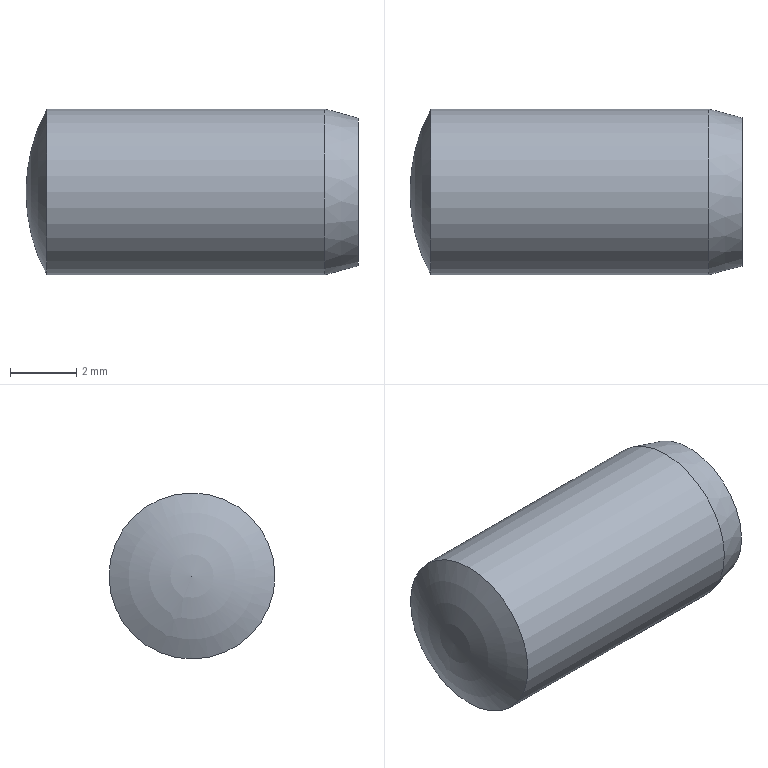Component | NX | CH3404_8-5_4 | 1 solid | 4 faces | box 10 x 5 x 5 mm | volume 188 mm3 | sphere 1 | plane 1 | cone 1 | cylinder 1 | commonest cylinder face diameters 5 x1
STEP:
#1=CARTESIAN_POINT('',(0.,0.,0.));
#2=DIRECTION('',(0.,0.,1.));
#3=DIRECTION('',(1.,0.,0.));
#4=AXIS2_PLACEMENT_3D('',#1,#2,#3);
#5=CARTESIAN_POINT('',(-39.37,0.9546,97.689));
#6=VERTEX_POINT('',#5);
#7=CARTESIAN_POINT('',(-39.37,-2.311,99.045));
#8=VERTEX_POINT('',#7);
#9=CARTESIAN_POINT('',(-39.37,0.,100.));
#10=DIRECTION('',(1.,0.,0.));
#11=DIRECTION('',(0.,-0.9242,-0.3818));
#12=AXIS2_PLACEMENT_3D('',#9,#10,#11);
#13=CIRCLE('',#12,2.5);
#14=CARTESIAN_POINT('',(-34.725,0.,100.));
#15=DIRECTION('',(1.,0.,0.));
#16=DIRECTION('',(-0.,0.3818,-0.9242));
#17=AXIS2_PLACEMENT_3D('',#14,#15,#16);
#18=SPHERICAL_SURFACE('',#17,5.275);
#19=CARTESIAN_POINT('',(-1.571,-1.077));
#20=CARTESIAN_POINT('',(-1.476,-1.077));
#21=CARTESIAN_POINT('',(-1.285,-1.077));
#22=CARTESIAN_POINT('',(-0.9996,-1.077));
#23=CARTESIAN_POINT('',(-0.714,-1.077));
#24=CARTESIAN_POINT('',(-0.4284,-1.077));
#25=CARTESIAN_POINT('',(-0.1428,-1.077));
#26=CARTESIAN_POINT('',(0.1428,-1.077));
#27=CARTESIAN_POINT('',(0.4284,-1.077));
#28=CARTESIAN_POINT('',(0.714,-1.077));
#29=CARTESIAN_POINT('',(0.9996,-1.077));
#30=CARTESIAN_POINT('',(1.285,-1.077));
#31=CARTESIAN_POINT('',(1.571,-1.077));
#32=CARTESIAN_POINT('',(1.856,-1.077));
#33=CARTESIAN_POINT('',(2.142,-1.077));
#34=CARTESIAN_POINT('',(2.428,-1.077));
#35=CARTESIAN_POINT('',(2.713,-1.077));
#36=CARTESIAN_POINT('',(2.999,-1.077));
#37=CARTESIAN_POINT('',(3.284,-1.077));
#38=CARTESIAN_POINT('',(3.57,-1.077));
#39=CARTESIAN_POINT('',(3.856,-1.077));
#40=CARTESIAN_POINT('',(4.141,-1.077));
#41=CARTESIAN_POINT('',(4.427,-1.077));
#42=CARTESIAN_POINT('',(4.617,-1.077));
#43=CARTESIAN_POINT('',(4.712,-1.077));
#44=B_SPLINE_CURVE_WITH_KNOTS('',3,(#19,#20,#21,#22,#23,#24,#25,#26,#27,#28,#29,#30,#31,#32,#33,#34,#35,#36,#37,#38,#39,#40,#41,#42,#43),.UNSPECIFIED.,.F.,.F.,(4,1,1,1,1,1,1,1,1,1,1,1,1,1,1,1,1,1,1,1,1,1,4),(0.,0.2856,0.5712,0.8568,1.142,1.428,1.714,1.999,2.285,2.57,2.856,3.142,3.427,3.713,3.998,4.284,4.57,4.855,5.141,5.426,5.712,5.998,6.283),.QUASI_UNIFORM_KNOTS.);
#45=(GEOMETRIC_REPRESENTATION_CONTEXT(2)PARAMETRIC_REPRESENTATION_CONTEXT()REPRESENTATION_CONTEXT('',''));
#46=DEFINITIONAL_REPRESENTATION('',(#44),#45);
#47=PCURVE('',#18,#46);
#48=CARTESIAN_POINT('',(-30.,0.,100.));
#49=DIRECTION('',(1.,0.,0.));
#50=DIRECTION('',(0.,-0.9242,-0.3818));
#51=AXIS2_PLACEMENT_3D('',#48,#49,#50);
#52=CYLINDRICAL_SURFACE('',#51,2.5);
#53=CARTESIAN_POINT('',(-0.,-9.37));
#54=DIRECTION('',(1.,0.));
#55=VECTOR('',#54,1.);
#56=LINE('',#53,#55);
#57=(GEOMETRIC_REPRESENTATION_CONTEXT(2)PARAMETRIC_REPRESENTATION_CONTEXT()REPRESENTATION_CONTEXT('',''));
#58=DEFINITIONAL_REPRESENTATION('',(#56),#57);
#59=PCURVE('',#52,#58);
#60=SURFACE_CURVE('',#13,(#47,#59),.PCURVE_S1.);
#61=EDGE_CURVE('',#6,#8,#60,.T.);
#62=ORIENTED_EDGE('',*,*,#61,.F.);
#63=CARTESIAN_POINT('',(-40.,-0.,100.));
#64=VERTEX_POINT('',#63);
#65=CARTESIAN_POINT('',(-40.,0.,100.));
#66=CARTESIAN_POINT('',(-40.,0.1989,99.519));
#67=CARTESIAN_POINT('',(-39.936,0.3978,99.037));
#68=CARTESIAN_POINT('',(-39.807,0.5927,98.565));
#69=CARTESIAN_POINT('',(-39.617,0.7795,98.113));
#70=CARTESIAN_POINT('',(-39.37,0.9546,97.689));
#71=B_SPLINE_CURVE_WITH_KNOTS('',5,(#65,#66,#67,#68,#69,#70),.UNSPECIFIED.,.F.,.F.,(6,6),(-1.571,-1.077),.PIECEWISE_BEZIER_KNOTS.);
#72=CARTESIAN_POINT('',(0.,0.));
#73=DIRECTION('',(0.,1.));
#74=VECTOR('',#73,1.);
#75=LINE('',#72,#74);
#76=(GEOMETRIC_REPRESENTATION_CONTEXT(2)PARAMETRIC_REPRESENTATION_CONTEXT()REPRESENTATION_CONTEXT('',''));
#77=DEFINITIONAL_REPRESENTATION('',(#75),#76);
#78=PCURVE('',#18,#77);
#79=CARTESIAN_POINT('',(6.283,0.));
#80=DIRECTION('',(0.,1.));
#81=VECTOR('',#80,1.);
#82=LINE('',#79,#81);
#83=(GEOMETRIC_REPRESENTATION_CONTEXT(2)PARAMETRIC_REPRESENTATION_CONTEXT()REPRESENTATION_CONTEXT('',''));
#84=DEFINITIONAL_REPRESENTATION('',(#82),#83);
#85=PCURVE('',#18,#84);
#86=SEAM_CURVE('',#71,(#78,#85),.PCURVE_S1.);
#87=EDGE_CURVE('',#64,#6,#86,.T.);
#88=ORIENTED_EDGE('',*,*,#87,.F.);
#89=ORIENTED_EDGE('',*,*,#87,.T.);
#90=CARTESIAN_POINT('',(-39.37,0.,100.));
#91=DIRECTION('',(1.,0.,0.));
#92=DIRECTION('',(0.,-0.9242,-0.3818));
#93=AXIS2_PLACEMENT_3D('',#90,#91,#92);
#94=CIRCLE('',#93,2.5);
#95=CARTESIAN_POINT('',(4.712,-1.077));
#96=CARTESIAN_POINT('',(4.808,-1.077));
#97=CARTESIAN_POINT('',(4.998,-1.077));
#98=CARTESIAN_POINT('',(5.284,-1.077));
#99=CARTESIAN_POINT('',(5.569,-1.077));
#100=CARTESIAN_POINT('',(5.855,-1.077));
#101=CARTESIAN_POINT('',(6.14,-1.077));
#102=CARTESIAN_POINT('',(6.426,-1.077));
#103=CARTESIAN_POINT('',(6.712,-1.077));
#104=CARTESIAN_POINT('',(6.997,-1.077));
#105=CARTESIAN_POINT('',(7.283,-1.077));
#106=CARTESIAN_POINT('',(7.568,-1.077));
#107=CARTESIAN_POINT('',(7.854,-1.077));
#108=CARTESIAN_POINT('',(8.14,-1.077));
#109=CARTESIAN_POINT('',(8.425,-1.077));
#110=CARTESIAN_POINT('',(8.711,-1.077));
#111=CARTESIAN_POINT('',(8.996,-1.077));
#112=CARTESIAN_POINT('',(9.282,-1.077));
#113=CARTESIAN_POINT('',(9.568,-1.077));
#114=CARTESIAN_POINT('',(9.853,-1.077));
#115=CARTESIAN_POINT('',(10.139,-1.077));
#116=CARTESIAN_POINT('',(10.424,-1.077));
#117=CARTESIAN_POINT('',(10.71,-1.077));
#118=CARTESIAN_POINT('',(10.9,-1.077));
#119=CARTESIAN_POINT('',(10.996,-1.077));
#120=B_SPLINE_CURVE_WITH_KNOTS('',3,(#95,#96,#97,#98,#99,#100,#101,#102,#103,#104,#105,#106,#107,#108,#109,#110,#111,#112,#113,#114,#115,#116,#117,#118,#119),.UNSPECIFIED.,.F.,.F.,(4,1,1,1,1,1,1,1,1,1,1,1,1,1,1,1,1,1,1,1,1,1,4),(0.,0.2856,0.5712,0.8568,1.142,1.428,1.714,1.999,2.285,2.57,2.856,3.142,3.427,3.713,3.998,4.284,4.57,4.855,5.141,5.426,5.712,5.998,6.283),.QUASI_UNIFORM_KNOTS.);
#121=(GEOMETRIC_REPRESENTATION_CONTEXT(2)PARAMETRIC_REPRESENTATION_CONTEXT()REPRESENTATION_CONTEXT('',''));
#122=DEFINITIONAL_REPRESENTATION('',(#120),#121);
#123=PCURVE('',#18,#122);
#124=CARTESIAN_POINT('',(0.,-9.37));
#125=DIRECTION('',(1.,0.));
#126=VECTOR('',#125,1.);
#127=LINE('',#124,#126);
#128=(GEOMETRIC_REPRESENTATION_CONTEXT(2)PARAMETRIC_REPRESENTATION_CONTEXT()REPRESENTATION_CONTEXT('',''));
#129=DEFINITIONAL_REPRESENTATION('',(#127),#128);
#130=PCURVE('',#52,#129);
#131=SURFACE_CURVE('',#94,(#123,#130),.PCURVE_S1.);
#132=EDGE_CURVE('',#8,#6,#131,.T.);
#133=ORIENTED_EDGE('',*,*,#132,.F.);
#134=EDGE_LOOP('',(#62,#88,#89,#133));
#135=FACE_BOUND('',#134,.T.);
#136=ADVANCED_FACE('',(#135),#18,.T.);
#137=CARTESIAN_POINT('',(-30.,-2.063,99.148));
#138=VERTEX_POINT('',#137);
#139=CARTESIAN_POINT('',(-30.,0.,100.));
#140=DIRECTION('',(1.,0.,0.));
#141=DIRECTION('',(0.,-0.9242,-0.3818));
#142=AXIS2_PLACEMENT_3D('',#139,#140,#141);
#143=CIRCLE('',#142,2.232);
#144=CARTESIAN_POINT('',(-30.,0.,100.));
#145=DIRECTION('',(1.,0.,0.));
#146=DIRECTION('',(0.,-0.9242,-0.3818));
#147=AXIS2_PLACEMENT_3D('',#144,#145,#146);
#148=PLANE('',#147);
#149=CARTESIAN_POINT('',(0.,-0.));
#150=DIRECTION('',(1.,0.));
#151=AXIS2_PLACEMENT_2D('',#149,#150);
#152=CIRCLE('',#151,2.232);
#153=(GEOMETRIC_REPRESENTATION_CONTEXT(2)PARAMETRIC_REPRESENTATION_CONTEXT()REPRESENTATION_CONTEXT('',''));
#154=DEFINITIONAL_REPRESENTATION('',(#152),#153);
#155=PCURVE('',#148,#154);
#156=CARTESIAN_POINT('',(-30.,0.,100.));
#157=DIRECTION('',(-1.,0.,0.));
#158=DIRECTION('',(0.,0.9242,0.3818));
#159=AXIS2_PLACEMENT_3D('',#156,#157,#158);
#160=CONICAL_SURFACE('',#159,2.232,0.2618);
#161=CARTESIAN_POINT('',(9.425,0.));
#162=DIRECTION('',(-1.,0.));
#163=VECTOR('',#162,1.);
#164=LINE('',#161,#163);
#165=(GEOMETRIC_REPRESENTATION_CONTEXT(2)PARAMETRIC_REPRESENTATION_CONTEXT()REPRESENTATION_CONTEXT('',''));
#166=DEFINITIONAL_REPRESENTATION('',(#164),#165);
#167=PCURVE('',#160,#166);
#168=SURFACE_CURVE('',#143,(#155,#167),.PCURVE_S1.);
#169=EDGE_CURVE('',#138,#138,#168,.T.);
#170=ORIENTED_EDGE('',*,*,#169,.T.);
#171=EDGE_LOOP('',(#170));
#172=FACE_BOUND('',#171,.T.);
#173=ADVANCED_FACE('',(#172),#148,.T.);
#174=CARTESIAN_POINT('',(-31.,-2.311,99.045));
#175=VERTEX_POINT('',#174);
#176=CARTESIAN_POINT('',(-31.,0.,100.));
#177=DIRECTION('',(1.,0.,0.));
#178=DIRECTION('',(0.,-0.9242,-0.3818));
#179=AXIS2_PLACEMENT_3D('',#176,#177,#178);
#180=CIRCLE('',#179,2.5);
#181=CARTESIAN_POINT('',(9.425,1.));
#182=DIRECTION('',(-1.,0.));
#183=VECTOR('',#182,1.);
#184=LINE('',#181,#183);
#185=(GEOMETRIC_REPRESENTATION_CONTEXT(2)PARAMETRIC_REPRESENTATION_CONTEXT()REPRESENTATION_CONTEXT('',''));
#186=DEFINITIONAL_REPRESENTATION('',(#184),#185);
#187=PCURVE('',#160,#186);
#188=CARTESIAN_POINT('',(0.,-1.));
#189=DIRECTION('',(1.,0.));
#190=VECTOR('',#189,1.);
#191=LINE('',#188,#190);
#192=(GEOMETRIC_REPRESENTATION_CONTEXT(2)PARAMETRIC_REPRESENTATION_CONTEXT()REPRESENTATION_CONTEXT('',''));
#193=DEFINITIONAL_REPRESENTATION('',(#191),#192);
#194=PCURVE('',#52,#193);
#195=SURFACE_CURVE('',#180,(#187,#194),.PCURVE_S1.);
#196=EDGE_CURVE('',#175,#175,#195,.T.);
#197=ORIENTED_EDGE('',*,*,#196,.T.);
#198=CARTESIAN_POINT('',(-30.,-2.063,99.148));
#199=CARTESIAN_POINT('',(-31.,-2.311,99.045));
#200=B_SPLINE_CURVE_WITH_KNOTS('',1,(#198,#199),.UNSPECIFIED.,.F.,.F.,(2,2),(0.,1.035),.PIECEWISE_BEZIER_KNOTS.);
#201=CARTESIAN_POINT('',(3.142,0.));
#202=DIRECTION('',(0.,1.));
#203=VECTOR('',#202,1.);
#204=LINE('',#201,#203);
#205=(GEOMETRIC_REPRESENTATION_CONTEXT(2)PARAMETRIC_REPRESENTATION_CONTEXT()REPRESENTATION_CONTEXT('',''));
#206=DEFINITIONAL_REPRESENTATION('',(#204),#205);
#207=PCURVE('',#160,#206);
#208=CARTESIAN_POINT('',(9.425,0.));
#209=DIRECTION('',(0.,1.));
#210=VECTOR('',#209,1.);
#211=LINE('',#208,#210);
#212=(GEOMETRIC_REPRESENTATION_CONTEXT(2)PARAMETRIC_REPRESENTATION_CONTEXT()REPRESENTATION_CONTEXT('',''));
#213=DEFINITIONAL_REPRESENTATION('',(#211),#212);
#214=PCURVE('',#160,#213);
#215=SEAM_CURVE('',#200,(#207,#214),.PCURVE_S1.);
#216=EDGE_CURVE('',#138,#175,#215,.T.);
#217=ORIENTED_EDGE('',*,*,#216,.F.);
#218=ORIENTED_EDGE('',*,*,#169,.F.);
#219=ORIENTED_EDGE('',*,*,#216,.T.);
#220=EDGE_LOOP('',(#197,#217,#218,#219));
#221=FACE_BOUND('',#220,.T.);
#222=ADVANCED_FACE('',(#221),#160,.T.);
#223=ORIENTED_EDGE('',*,*,#132,.T.);
#224=ORIENTED_EDGE('',*,*,#61,.T.);
#225=CARTESIAN_POINT('',(-39.37,-2.311,99.045));
#226=CARTESIAN_POINT('',(-31.,-2.311,99.045));
#227=B_SPLINE_CURVE_WITH_KNOTS('',1,(#225,#226),.UNSPECIFIED.,.F.,.F.,(2,2),(-9.37,-1.),.PIECEWISE_BEZIER_KNOTS.);
#228=CARTESIAN_POINT('',(6.283,0.));
#229=DIRECTION('',(0.,1.));
#230=VECTOR('',#229,1.);
#231=LINE('',#228,#230);
#232=(GEOMETRIC_REPRESENTATION_CONTEXT(2)PARAMETRIC_REPRESENTATION_CONTEXT()REPRESENTATION_CONTEXT('',''));
#233=DEFINITIONAL_REPRESENTATION('',(#231),#232);
#234=PCURVE('',#52,#233);
#235=CARTESIAN_POINT('',(-0.,0.));
#236=DIRECTION('',(0.,1.));
#237=VECTOR('',#236,1.);
#238=LINE('',#235,#237);
#239=(GEOMETRIC_REPRESENTATION_CONTEXT(2)PARAMETRIC_REPRESENTATION_CONTEXT()REPRESENTATION_CONTEXT('',''));
#240=DEFINITIONAL_REPRESENTATION('',(#238),#239);
#241=PCURVE('',#52,#240);
#242=SEAM_CURVE('',#227,(#234,#241),.PCURVE_S1.);
#243=EDGE_CURVE('',#8,#175,#242,.T.);
#244=ORIENTED_EDGE('',*,*,#243,.T.);
#245=ORIENTED_EDGE('',*,*,#196,.F.);
#246=ORIENTED_EDGE('',*,*,#243,.F.);
#247=EDGE_LOOP('',(#223,#224,#244,#245,#246));
#248=FACE_BOUND('',#247,.T.);
#249=ADVANCED_FACE('',(#248),#52,.T.);
#250=CLOSED_SHELL('',(#136,#173,#222,#249));
#251=MANIFOLD_SOLID_BREP('',#250);
#252=(LENGTH_UNIT()NAMED_UNIT(*)SI_UNIT(.MILLI.,.METRE.));
#253=UNCERTAINTY_MEASURE_WITH_UNIT(LENGTH_MEASURE(0.00001),#252,'','');
#254=(NAMED_UNIT(*)PLANE_ANGLE_UNIT()SI_UNIT($,.RADIAN.));
#255=(NAMED_UNIT(*)SI_UNIT($,.STERADIAN.)SOLID_ANGLE_UNIT());
#256=(GEOMETRIC_REPRESENTATION_CONTEXT(3)GLOBAL_UNCERTAINTY_ASSIGNED_CONTEXT((#253))GLOBAL_UNIT_ASSIGNED_CONTEXT((#252,#254,#255))REPRESENTATION_CONTEXT('',''));
#257=ADVANCED_BREP_SHAPE_REPRESENTATION('',(#4,#251),#256);